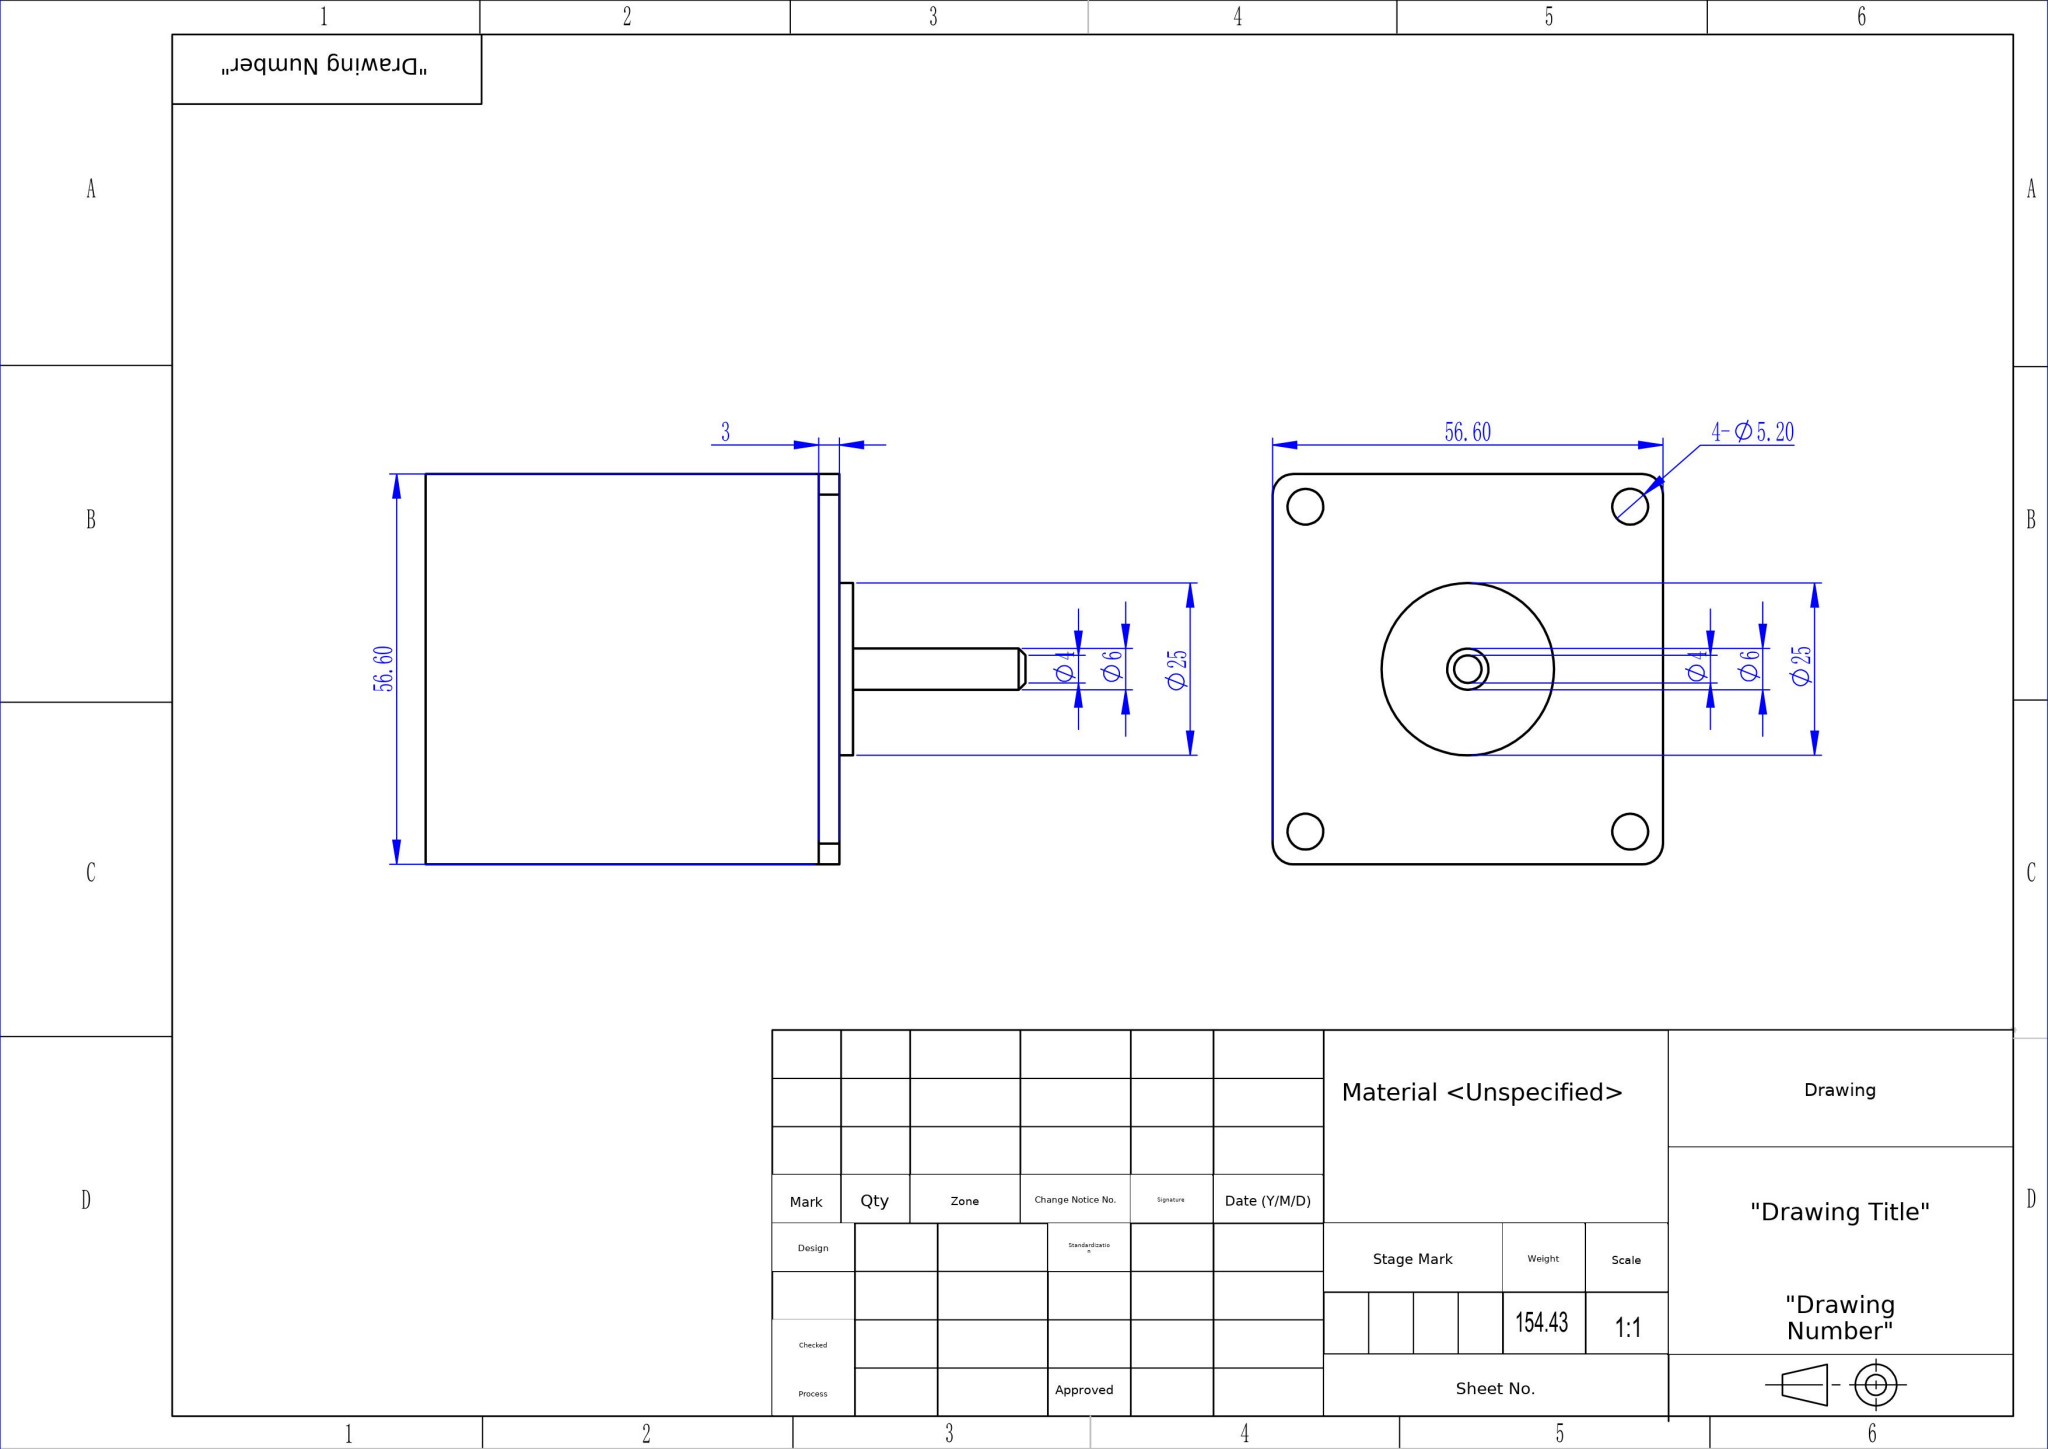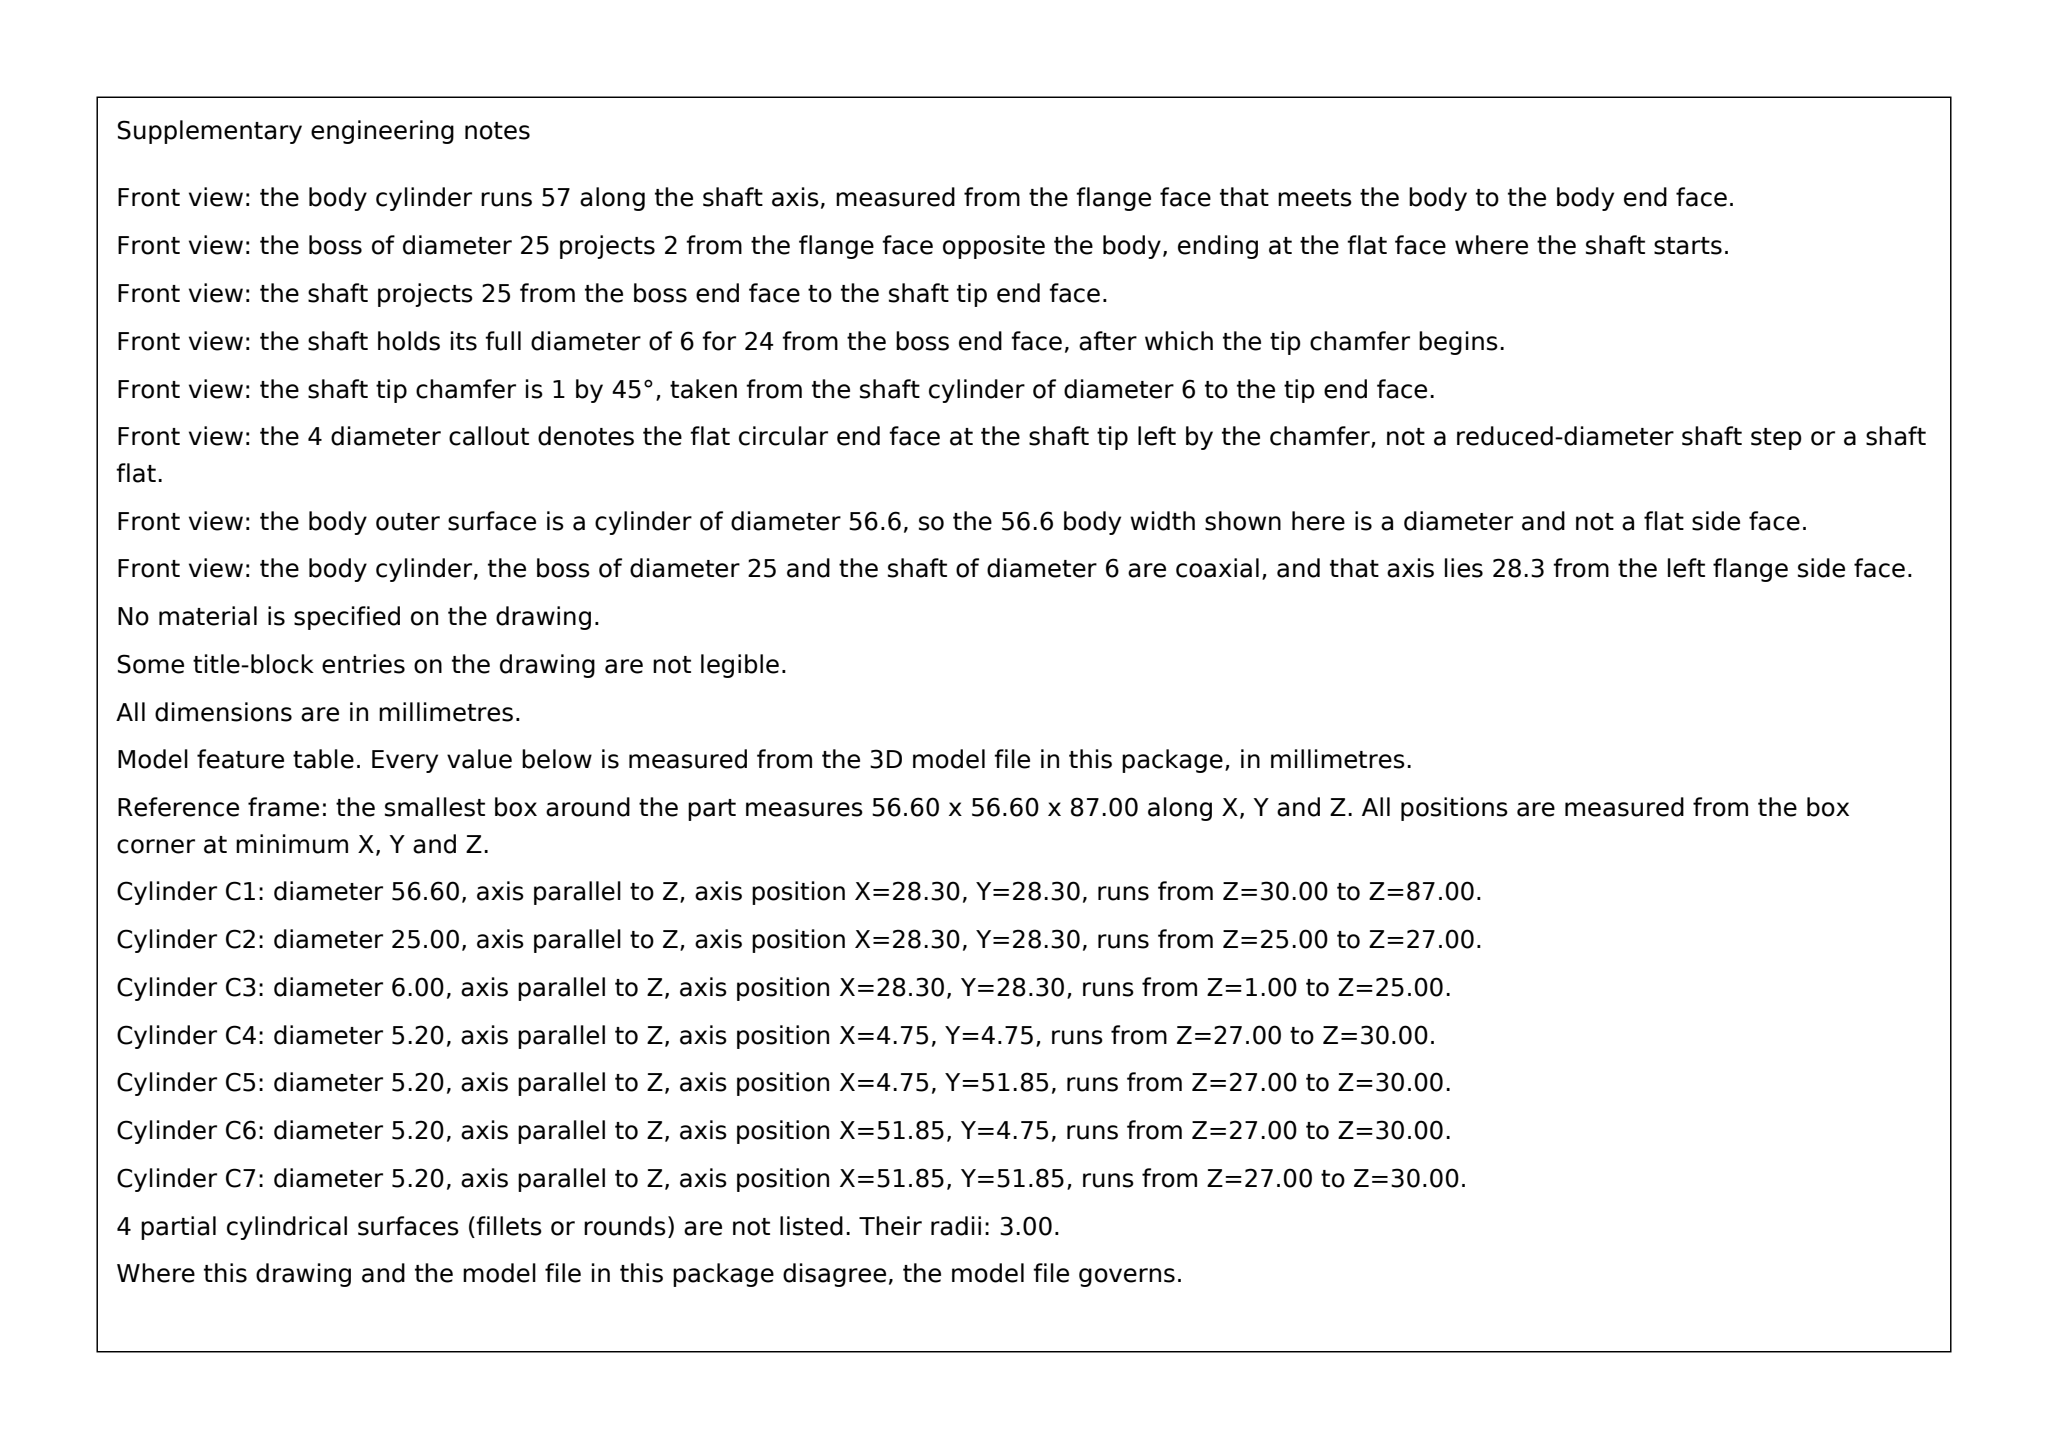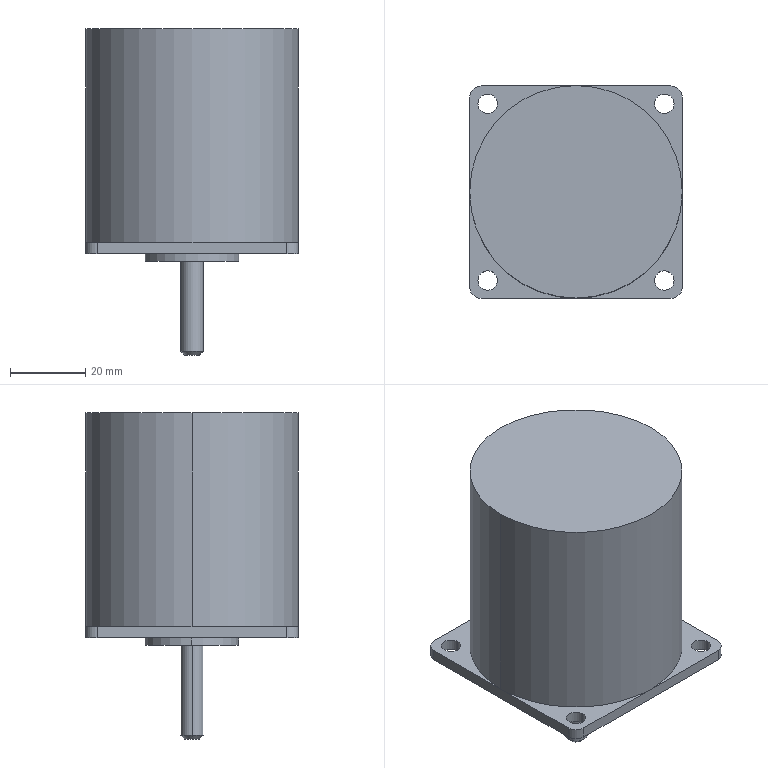Part | SolidWorks | mm | 1 solid | 32 faces | box 56.6 x 56.6 x 87 mm | volume 154429 mm3 | cylinder 18 | plane 12 | cone 2 | commonest cylinder face diameters 5.2 x8 6 x6 56.6 x2 25 x2
Drawing notes:
OVERALL LENGTH 87 FROM SHAFT END FACE TO REAR FACE OF BODY | from the solid: bbox_xyz z = 87.0; planes z=0.0 and z=87.0
MOTOR BODY LENGTH 57, MEASURED FROM FRONT FLANGE FACE (DATUM A, z=30) TO REAR FACE | from the solid: cylinder [56.6, z, (28.3,28.3), length 57] between planes z=30.0 and z=87.0
SHAFT Ø6 PROJECTS 24 FROM Ø25 BOSS FACE | from the solid: cylinder [6.0, z, (28.3,28.3), length 24.0] starting at plane z=25.0
BOSS Ø25 x 2 HIGH FROM FRONT FLANGE FACE (DATUM A) | from the solid: cylinder [25.0, z, (28.3,28.3), length 2.0] between planes z=25.0 and z=27.0
4X Ø5.20 THRU FLANGE, HOLE CENTRES 47.10 x 47.10 APART, 4.75 FROM EACH SIDE FACE | from the solid: cylinders 5.2 dia at (4.75,4.75), (4.75,51.85), (51.85,4.75), (51.85,51.85); side planes x=0/56.6, y=0/56.6
FOUR CORNERS OF FLANGE R3 (CENTRES 3 FROM EACH SIDE FACE) | from the solid: Ø6.0 z-cylinders length 3.0 at (3,3), (3,53.6), (53.6,3), (53.6,53.6) with side planes at 0 and 56.6
SHAFT END CHAMFER 90° INCLUDED ANGLE, Ø6 TO Ø4, 1 AXIAL AT SHAFT END FACE (z=0) | from the solid: cones [included_angle 90.0, ref_dia 4.0] on Ø6 shaft, plane z=0.0
build123d program:
from build123d import *

# Parameters (mm, degrees)
SKETCH1_R           = 2.6
BOSS_EXTRUDE1_DEPTH = 3
SKETCH2_R           = 12.5
BOSS_EXTRUDE2_DEPTH = 2
SKETCH3_R           = 28.3
BOSS_EXTRUDE3_DEPTH = 57
SKETCH4_R           = 3
BOSS_EXTRUDE4_DEPTH = 25
CHAMFER1_SIZE       = 1


with BuildPart() as part:
    # Sketch1 → Boss-Extrude1 (new body)
    with BuildSketch(Plane.XY):
        with BuildLine():
            Line((-25.3, 28.3), (25.3, 28.3))
            ThreePointArc((25.3, 28.3), (27.421, 27.421), (28.3, 25.3))
            Line((28.3, 25.3), (28.3, -25.3))
            ThreePointArc((28.3, -25.3), (27.421, -27.421), (25.3, -28.3))
            Line((25.3, -28.3), (-25.3, -28.3))
            ThreePointArc((-25.3, -28.3), (-27.421, -27.421), (-28.3, -25.3))
            Line((-28.3, -25.3), (-28.3, 25.3))
            ThreePointArc((-28.3, 25.3), (-27.421, 27.421), (-25.3, 28.3))
        make_face()
        with Locations((-23.55, 23.55)):
            Circle(SKETCH1_R, mode=Mode.SUBTRACT)
        with Locations(Location((23.55, 23.55, 0), (0, 0, 180))):
            Circle(SKETCH1_R, mode=Mode.SUBTRACT)
        with Locations((23.55, -23.55)):
            Circle(SKETCH1_R, mode=Mode.SUBTRACT)
        with Locations(Location((-23.55, -23.55, 0), (0, 0, 180))):
            Circle(SKETCH1_R, mode=Mode.SUBTRACT)
    extrude(amount=BOSS_EXTRUDE1_DEPTH)

    # Sketch2 → Boss-Extrude2 (add)
    with BuildSketch(Plane(origin=(0, 0, 0), x_dir=(-1, 0, 0), z_dir=(0, 0, -1))):
        Circle(SKETCH2_R)
    extrude(amount=BOSS_EXTRUDE2_DEPTH)

    # Sketch3 → Boss-Extrude3 (add)
    with BuildSketch(Plane.XY.offset(3)):
        Circle(SKETCH3_R)
    extrude(amount=BOSS_EXTRUDE3_DEPTH)

    # Sketch4 → Boss-Extrude4 (add)
    with BuildSketch(Plane(origin=(0, 0, -2), x_dir=(-1, 0, 0), z_dir=(0, 0, -1))):
        Circle(SKETCH4_R)
    extrude(amount=BOSS_EXTRUDE4_DEPTH)

    # Chamfer1
    chamfer1_edges = [part.edges().sort_by_distance(p)[0] for p in [
        (3, 0, -27),
    ]]
    chamfer(chamfer1_edges, length=CHAMFER1_SIZE)


solid = part.part